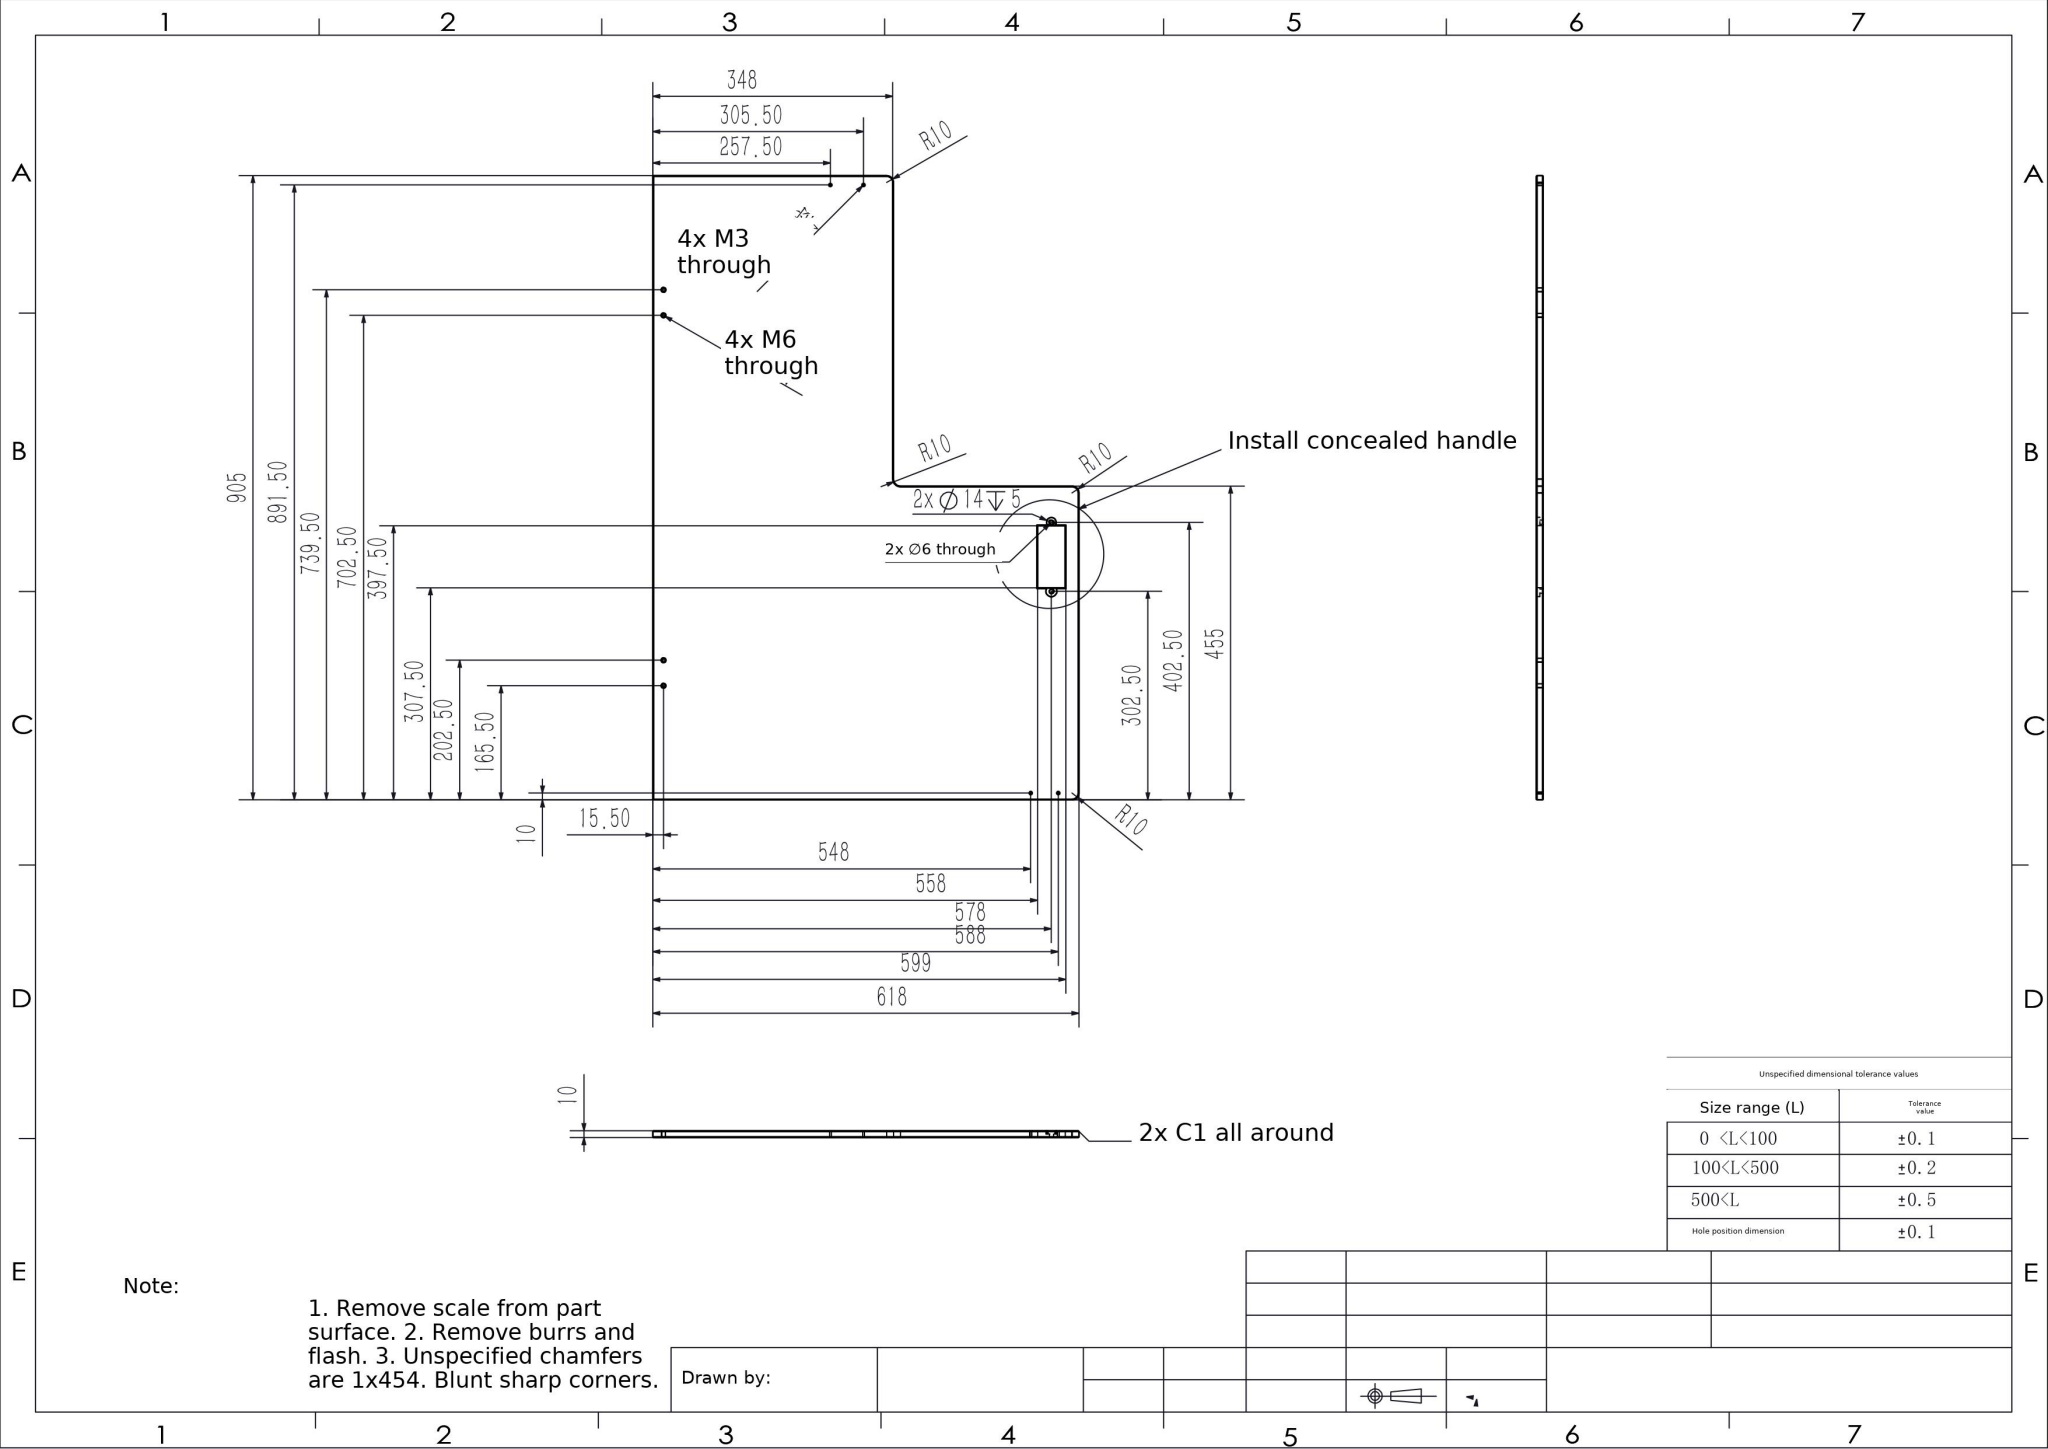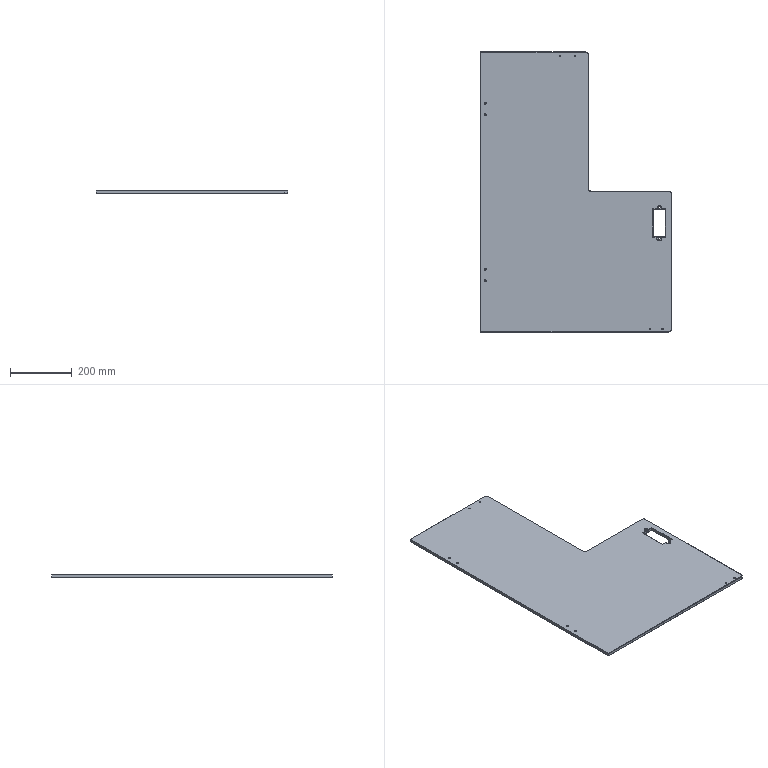Part | SolidWorks | mm | 1 solid | 110 faces | box 618 x 905 x 10 mm | volume 4339720 mm3 | cone 44 | plane 36 | cylinder 30 | commonest cylinder face diameters 2.5 x8 5 x8 6 x4 20 x4 14 x3 16 x3